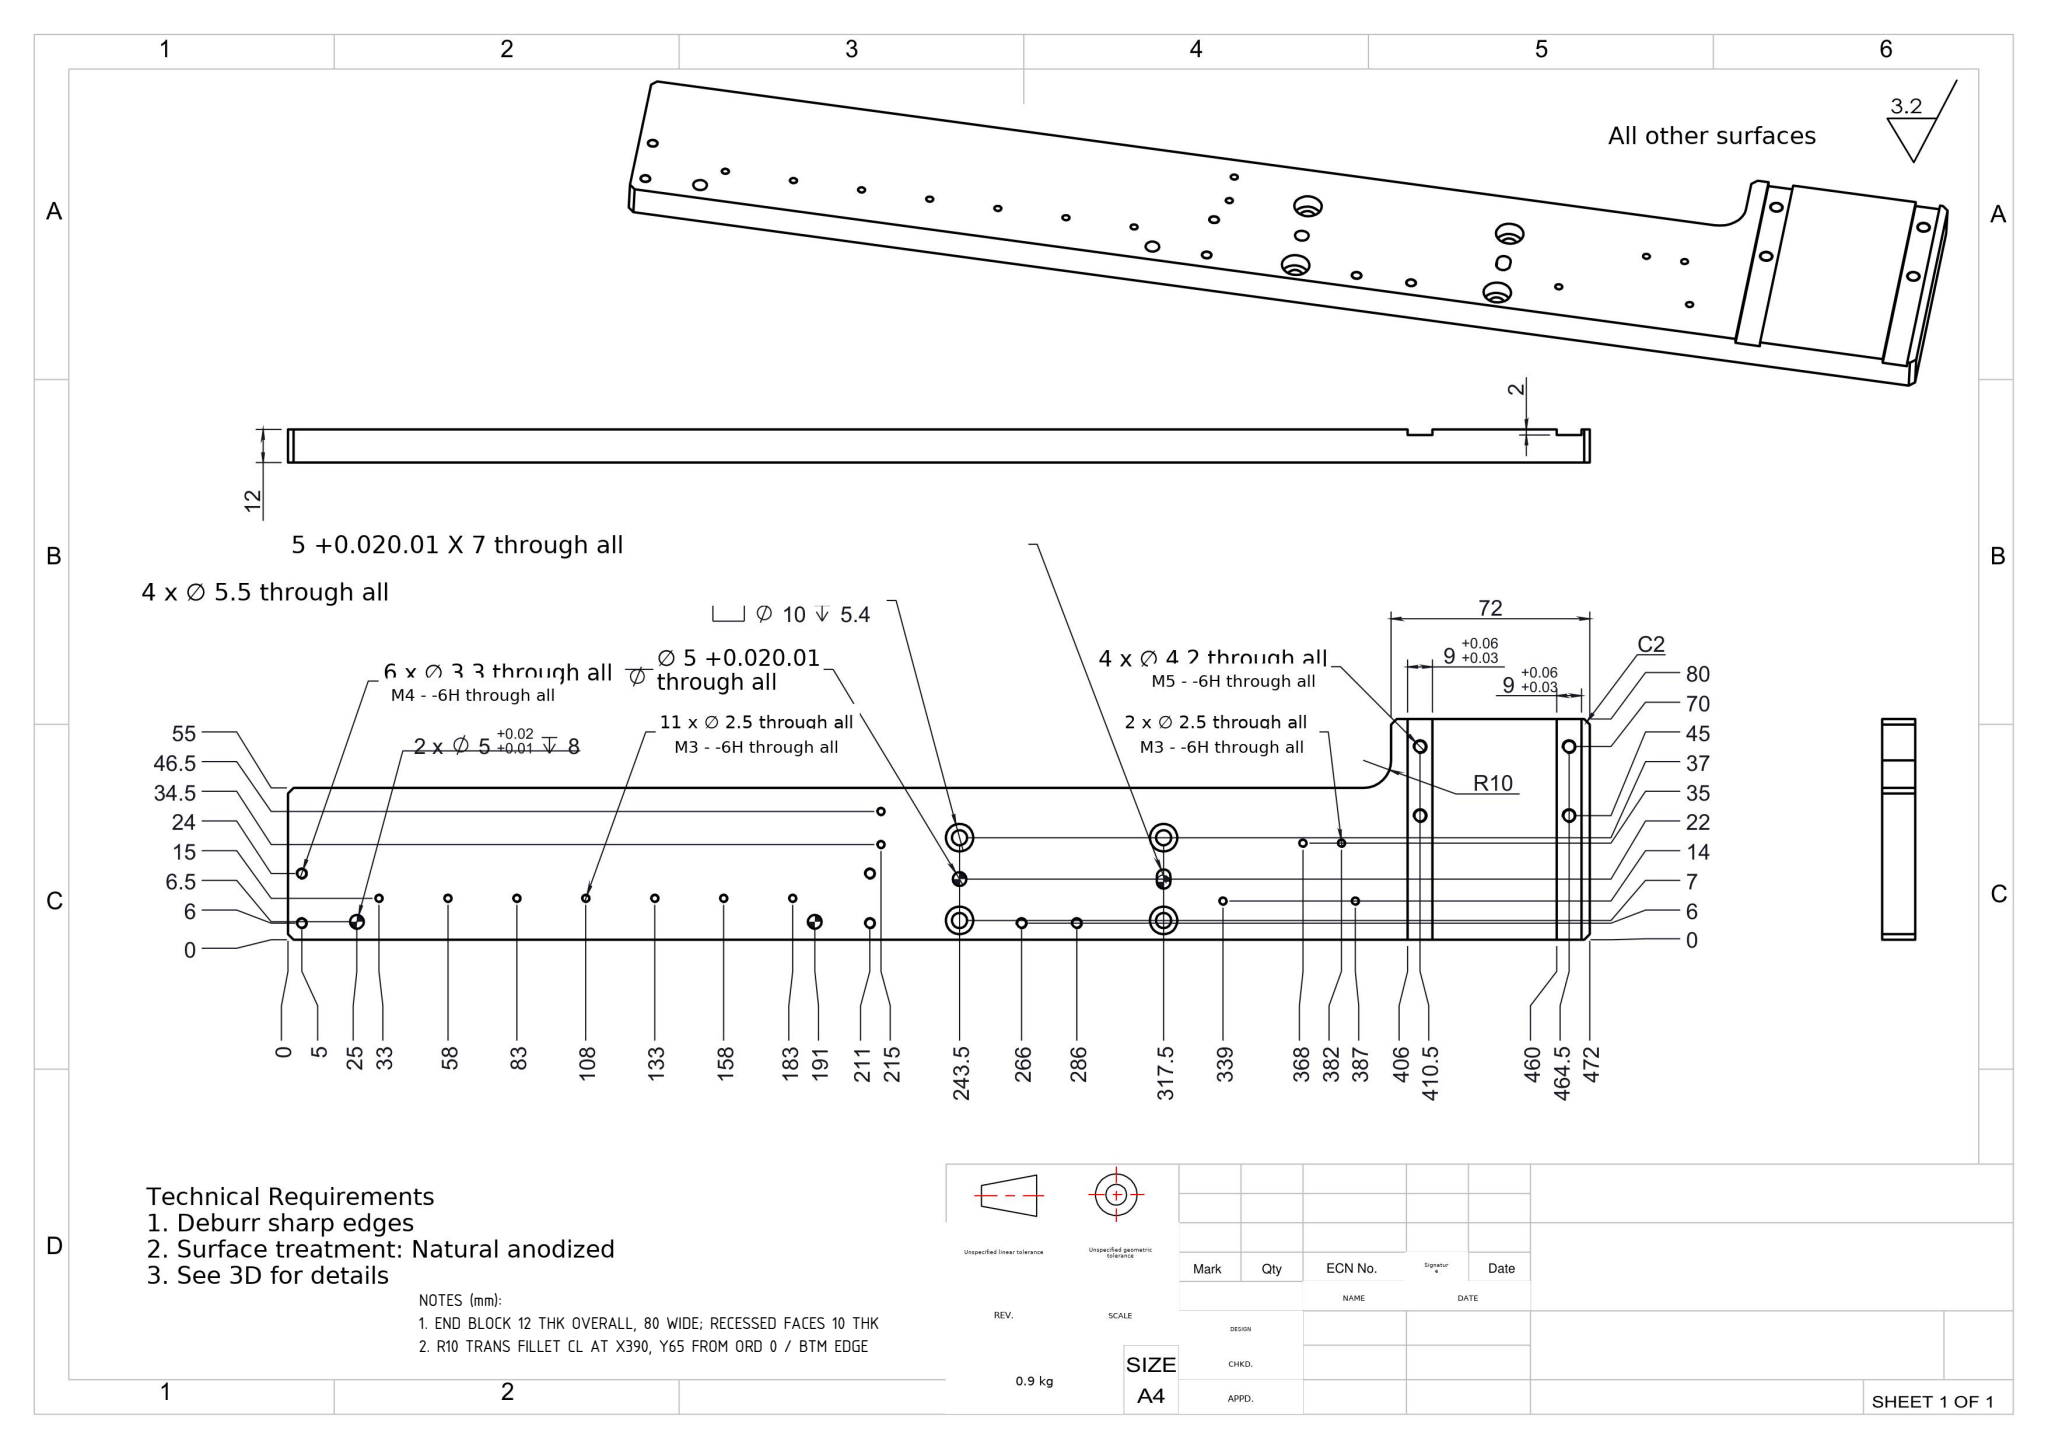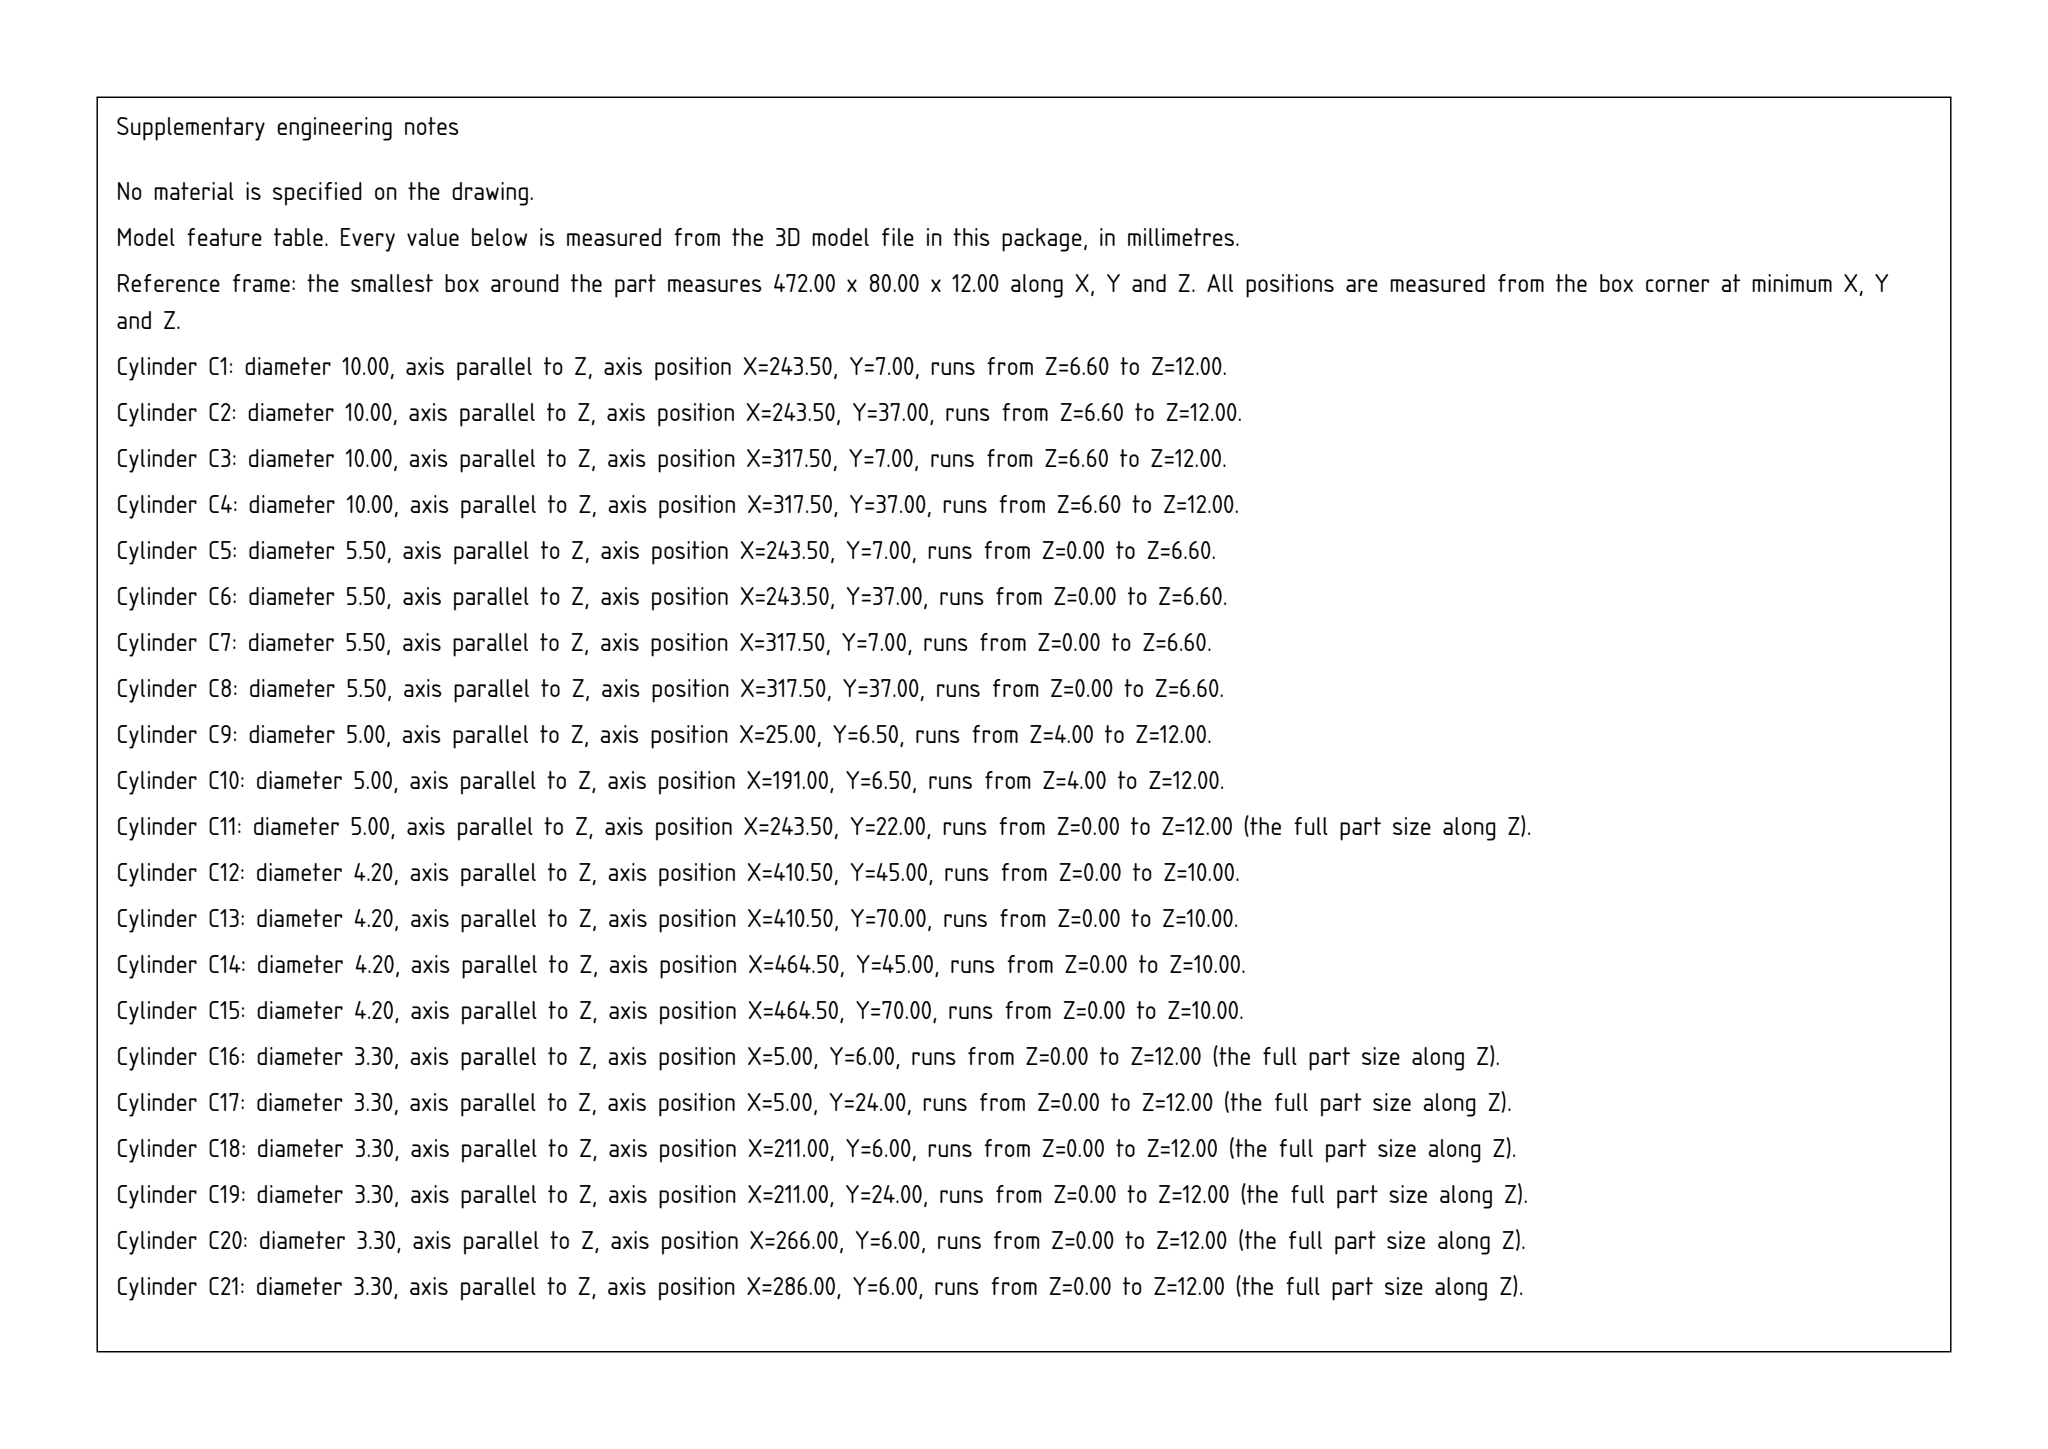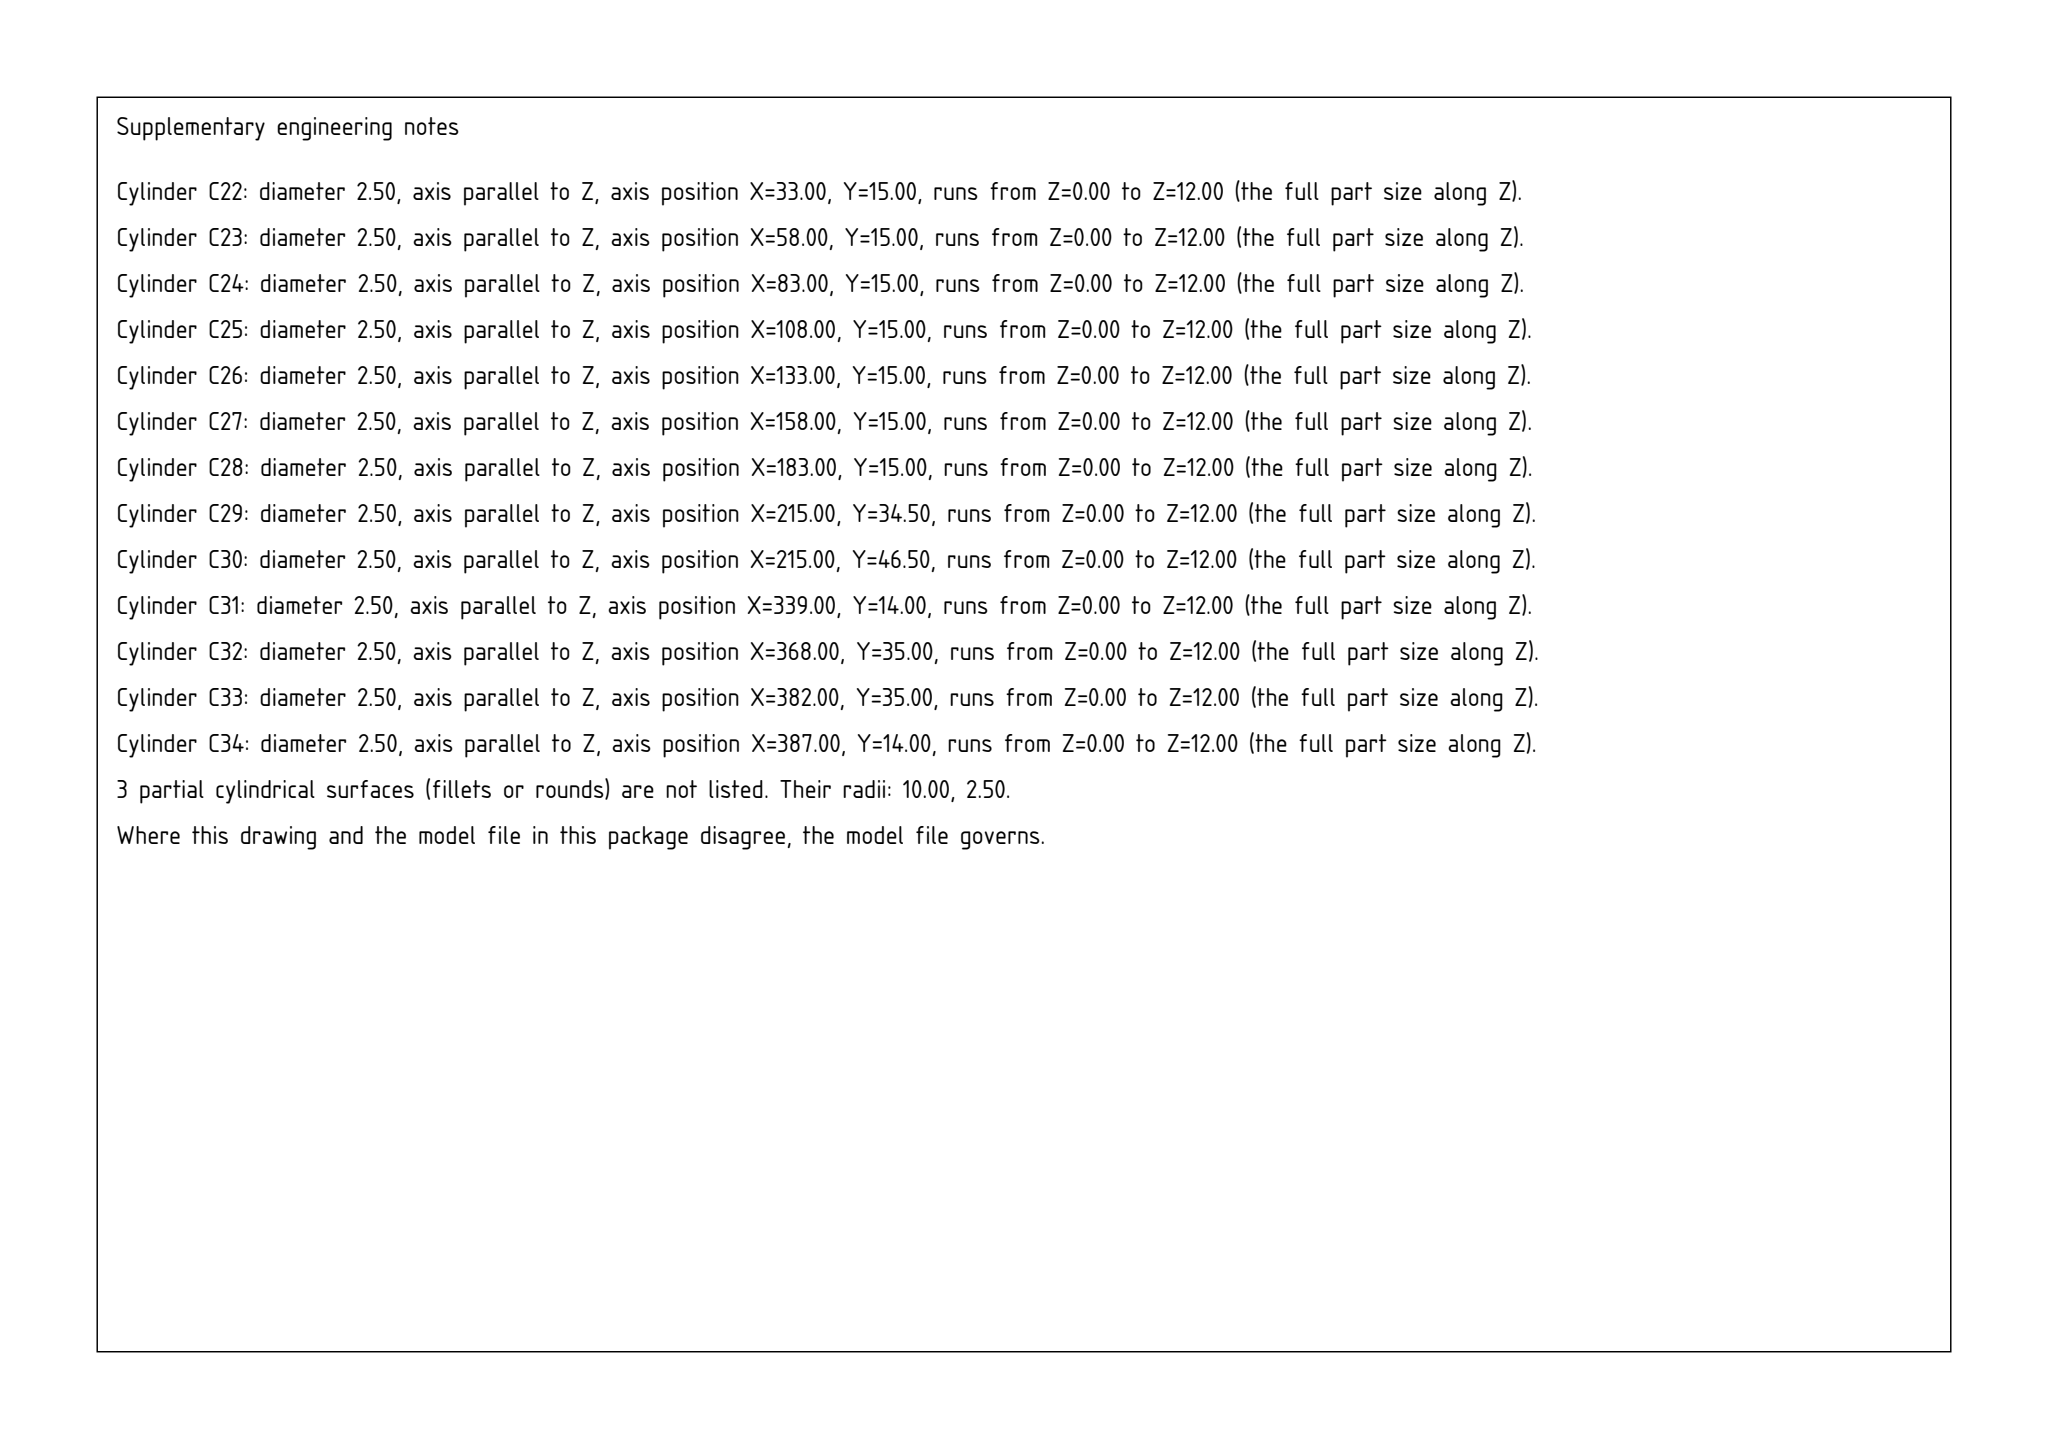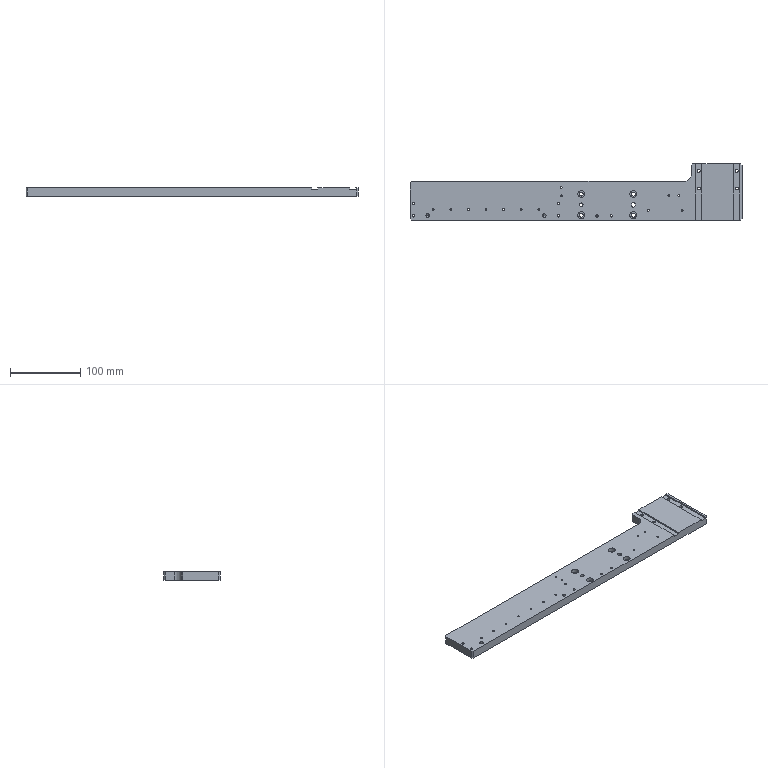Part | SolidWorks | mm | 1 solid | 102 faces | box 472 x 80 x 12 mm | volume 325193 mm3 | cylinder 71 | plane 27 | cone 4 | commonest cylinder face diameters 2.5 x26 3.3 x12 5 x8 4.2 x8 10 x8 5.5 x8 20 x1
Drawing notes:
END BLOCK 12 THK OVERALL, 80 WIDE; RECESSED FACES 10 THK | from the solid: bbox z=12; y planes 0/55/80; z plane 10 (2) under the 9-wide strips; Ø4.2 holes len 10
R10 TRANS FILLET CL AT X390, Y65 FROM ORD 0 / BTM EDGE | from the solid: Ø20 z-cylinder at (390,65) len 12, tangent to y=55 bar face and x=400 boss face